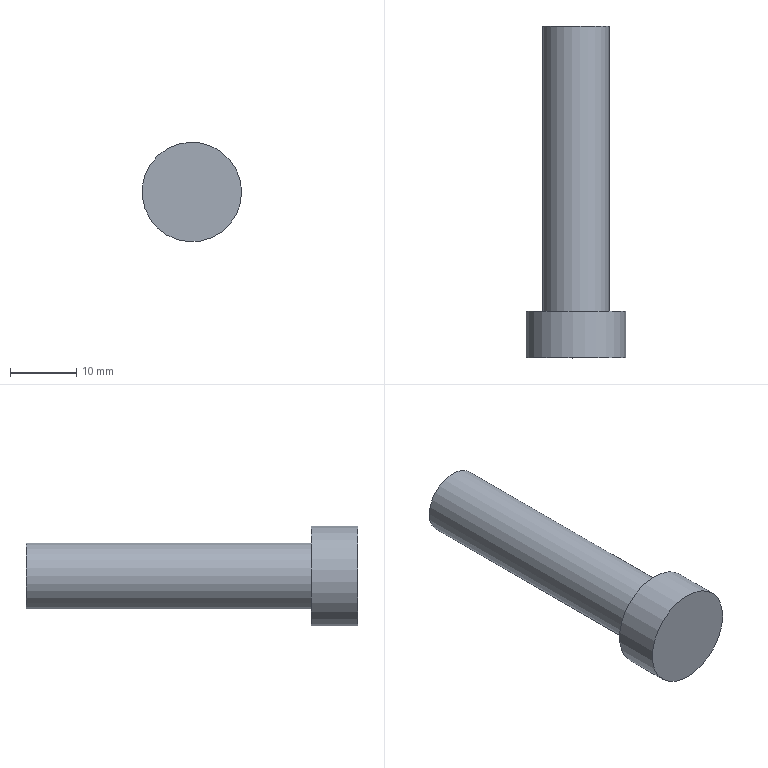Component | NX | LINK_PIN | 1 solid | 5 faces | box 15 x 50 x 15 mm | volume 4614 mm3 | plane 3 | cylinder 2 | commonest cylinder face diameters 10 x1 15 x1
STEP:
#1=CARTESIAN_POINT('',(0.,0.,0.));
#2=DIRECTION('',(0.,0.,1.));
#3=DIRECTION('',(1.,0.,0.));
#4=AXIS2_PLACEMENT_3D('',#1,#2,#3);
#5=CARTESIAN_POINT('',(12.507,-21.,-41.972));
#6=VERTEX_POINT('',#5);
#7=CARTESIAN_POINT('',(17.507,-21.,-41.994));
#8=DIRECTION('',(0.,-1.,0.));
#9=DIRECTION('',(-1.,0.,0.00428));
#10=AXIS2_PLACEMENT_3D('',#7,#8,#9);
#11=CIRCLE('',#10,5.);
#12=CARTESIAN_POINT('',(17.507,-28.,-41.994));
#13=DIRECTION('',(0.,1.,0.));
#14=DIRECTION('',(-1.,0.,0.00428));
#15=AXIS2_PLACEMENT_3D('',#12,#13,#14);
#16=CYLINDRICAL_SURFACE('',#15,5.);
#17=CARTESIAN_POINT('',(6.283,7.));
#18=DIRECTION('',(-1.,0.));
#19=VECTOR('',#18,1.);
#20=LINE('',#17,#19);
#21=(GEOMETRIC_REPRESENTATION_CONTEXT(2)PARAMETRIC_REPRESENTATION_CONTEXT()REPRESENTATION_CONTEXT('',''));
#22=DEFINITIONAL_REPRESENTATION('',(#20),#21);
#23=PCURVE('',#16,#22);
#24=CARTESIAN_POINT('',(17.507,-21.,-41.994));
#25=DIRECTION('',(0.,1.,0.));
#26=DIRECTION('',(-1.,0.,0.00428));
#27=AXIS2_PLACEMENT_3D('',#24,#25,#26);
#28=PLANE('',#27);
#29=CARTESIAN_POINT('',(5.,-0.));
#30=CARTESIAN_POINT('',(5.,-8.66));
#31=CARTESIAN_POINT('',(-2.5,-4.33));
#32=CARTESIAN_POINT('',(-10.,-0.));
#33=CARTESIAN_POINT('',(-2.5,4.33));
#34=CARTESIAN_POINT('',(5.,8.66));
#35=CARTESIAN_POINT('',(5.,-0.));
#36=(BOUNDED_CURVE()B_SPLINE_CURVE(2,(#29,#30,#31,#32,#33,#34,#35),.UNSPECIFIED.,.T.,.F.)B_SPLINE_CURVE_WITH_KNOTS((1,2,2,2,2,1),(-2.094,0.,2.094,4.189,6.283,8.378),.UNSPECIFIED.)CURVE()GEOMETRIC_REPRESENTATION_ITEM()RATIONAL_B_SPLINE_CURVE((1.,0.5,1.,0.5,1.,0.5,1.))REPRESENTATION_ITEM(''));
#37=(GEOMETRIC_REPRESENTATION_CONTEXT(2)PARAMETRIC_REPRESENTATION_CONTEXT()REPRESENTATION_CONTEXT('',''));
#38=DEFINITIONAL_REPRESENTATION('',(#36),#37);
#39=PCURVE('',#28,#38);
#40=SURFACE_CURVE('',#11,(#23,#39),.PCURVE_S1.);
#41=EDGE_CURVE('',#6,#6,#40,.T.);
#42=ORIENTED_EDGE('',*,*,#41,.F.);
#43=CARTESIAN_POINT('',(12.507,22.,-41.972));
#44=VERTEX_POINT('',#43);
#45=CARTESIAN_POINT('',(12.507,-21.,-41.972));
#46=CARTESIAN_POINT('',(12.507,22.,-41.972));
#47=B_SPLINE_CURVE_WITH_KNOTS('',1,(#45,#46),.UNSPECIFIED.,.F.,.F.,(2,2),(7.,50.),.PIECEWISE_BEZIER_KNOTS.);
#48=CARTESIAN_POINT('',(6.283,0.));
#49=DIRECTION('',(0.,1.));
#50=VECTOR('',#49,1.);
#51=LINE('',#48,#50);
#52=(GEOMETRIC_REPRESENTATION_CONTEXT(2)PARAMETRIC_REPRESENTATION_CONTEXT()REPRESENTATION_CONTEXT('',''));
#53=DEFINITIONAL_REPRESENTATION('',(#51),#52);
#54=PCURVE('',#16,#53);
#55=CARTESIAN_POINT('',(0.,0.));
#56=DIRECTION('',(0.,1.));
#57=VECTOR('',#56,1.);
#58=LINE('',#55,#57);
#59=(GEOMETRIC_REPRESENTATION_CONTEXT(2)PARAMETRIC_REPRESENTATION_CONTEXT()REPRESENTATION_CONTEXT('',''));
#60=DEFINITIONAL_REPRESENTATION('',(#58),#59);
#61=PCURVE('',#16,#60);
#62=SEAM_CURVE('',#47,(#54,#61),.PCURVE_S1.);
#63=EDGE_CURVE('',#6,#44,#62,.T.);
#64=ORIENTED_EDGE('',*,*,#63,.T.);
#65=CARTESIAN_POINT('',(22.506,22.,-42.015));
#66=VERTEX_POINT('',#65);
#67=CARTESIAN_POINT('',(17.507,22.,-41.994));
#68=DIRECTION('',(0.,1.,0.));
#69=DIRECTION('',(1.,0.,-0.00428));
#70=AXIS2_PLACEMENT_3D('',#67,#68,#69);
#71=CIRCLE('',#70,5.);
#72=CARTESIAN_POINT('',(3.142,50.));
#73=DIRECTION('',(1.,0.));
#74=VECTOR('',#73,1.);
#75=LINE('',#72,#74);
#76=(GEOMETRIC_REPRESENTATION_CONTEXT(2)PARAMETRIC_REPRESENTATION_CONTEXT()REPRESENTATION_CONTEXT('',''));
#77=DEFINITIONAL_REPRESENTATION('',(#75),#76);
#78=PCURVE('',#16,#77);
#79=CARTESIAN_POINT('',(17.507,22.,-41.994));
#80=DIRECTION('',(0.,1.,0.));
#81=DIRECTION('',(-1.,0.,0.00428));
#82=AXIS2_PLACEMENT_3D('',#79,#80,#81);
#83=PLANE('',#82);
#84=CARTESIAN_POINT('',(0.,0.));
#85=DIRECTION('',(-1.,0.));
#86=AXIS2_PLACEMENT_2D('',#84,#85);
#87=CIRCLE('',#86,5.);
#88=(GEOMETRIC_REPRESENTATION_CONTEXT(2)PARAMETRIC_REPRESENTATION_CONTEXT()REPRESENTATION_CONTEXT('',''));
#89=DEFINITIONAL_REPRESENTATION('',(#87),#88);
#90=PCURVE('',#83,#89);
#91=SURFACE_CURVE('',#71,(#78,#90),.PCURVE_S1.);
#92=EDGE_CURVE('',#66,#44,#91,.T.);
#93=ORIENTED_EDGE('',*,*,#92,.F.);
#94=CARTESIAN_POINT('',(17.507,22.,-41.994));
#95=DIRECTION('',(0.,1.,0.));
#96=DIRECTION('',(1.,0.,-0.00428));
#97=AXIS2_PLACEMENT_3D('',#94,#95,#96);
#98=CIRCLE('',#97,5.);
#99=CARTESIAN_POINT('',(-3.142,50.));
#100=DIRECTION('',(1.,0.));
#101=VECTOR('',#100,1.);
#102=LINE('',#99,#101);
#103=(GEOMETRIC_REPRESENTATION_CONTEXT(2)PARAMETRIC_REPRESENTATION_CONTEXT()REPRESENTATION_CONTEXT('',''));
#104=DEFINITIONAL_REPRESENTATION('',(#102),#103);
#105=PCURVE('',#16,#104);
#106=CARTESIAN_POINT('',(0.,0.));
#107=DIRECTION('',(-1.,0.));
#108=AXIS2_PLACEMENT_2D('',#106,#107);
#109=CIRCLE('',#108,5.);
#110=(GEOMETRIC_REPRESENTATION_CONTEXT(2)PARAMETRIC_REPRESENTATION_CONTEXT()REPRESENTATION_CONTEXT('',''));
#111=DEFINITIONAL_REPRESENTATION('',(#109),#110);
#112=PCURVE('',#83,#111);
#113=SURFACE_CURVE('',#98,(#105,#112),.PCURVE_S1.);
#114=EDGE_CURVE('',#44,#66,#113,.T.);
#115=ORIENTED_EDGE('',*,*,#114,.F.);
#116=ORIENTED_EDGE('',*,*,#63,.F.);
#117=EDGE_LOOP('',(#42,#64,#93,#115,#116));
#118=FACE_BOUND('',#117,.T.);
#119=ADVANCED_FACE('',(#118),#16,.T.);
#120=ORIENTED_EDGE('',*,*,#92,.T.);
#121=ORIENTED_EDGE('',*,*,#114,.T.);
#122=EDGE_LOOP('',(#120,#121));
#123=FACE_BOUND('',#122,.T.);
#124=ADVANCED_FACE('',(#123),#83,.T.);
#125=CARTESIAN_POINT('',(25.006,-28.,-42.026));
#126=VERTEX_POINT('',#125);
#127=CARTESIAN_POINT('',(17.507,-28.,-41.994));
#128=DIRECTION('',(0.,1.,0.));
#129=DIRECTION('',(1.,0.,-0.00428));
#130=AXIS2_PLACEMENT_3D('',#127,#128,#129);
#131=CIRCLE('',#130,7.5);
#132=CARTESIAN_POINT('',(17.507,-28.,-41.994));
#133=DIRECTION('',(0.,1.,0.));
#134=DIRECTION('',(-1.,0.,0.00428));
#135=AXIS2_PLACEMENT_3D('',#132,#133,#134);
#136=CYLINDRICAL_SURFACE('',#135,7.5);
#137=CARTESIAN_POINT('',(3.142,0.));
#138=DIRECTION('',(1.,0.));
#139=VECTOR('',#138,1.);
#140=LINE('',#137,#139);
#141=(GEOMETRIC_REPRESENTATION_CONTEXT(2)PARAMETRIC_REPRESENTATION_CONTEXT()REPRESENTATION_CONTEXT('',''));
#142=DEFINITIONAL_REPRESENTATION('',(#140),#141);
#143=PCURVE('',#136,#142);
#144=CARTESIAN_POINT('',(17.507,-28.,-41.994));
#145=DIRECTION('',(0.,1.,0.));
#146=DIRECTION('',(-1.,0.,0.00428));
#147=AXIS2_PLACEMENT_3D('',#144,#145,#146);
#148=PLANE('',#147);
#149=CARTESIAN_POINT('',(0.,0.));
#150=DIRECTION('',(-1.,0.));
#151=AXIS2_PLACEMENT_2D('',#149,#150);
#152=CIRCLE('',#151,7.5);
#153=(GEOMETRIC_REPRESENTATION_CONTEXT(2)PARAMETRIC_REPRESENTATION_CONTEXT()REPRESENTATION_CONTEXT('',''));
#154=DEFINITIONAL_REPRESENTATION('',(#152),#153);
#155=PCURVE('',#148,#154);
#156=SURFACE_CURVE('',#131,(#143,#155),.PCURVE_S1.);
#157=EDGE_CURVE('',#126,#126,#156,.T.);
#158=ORIENTED_EDGE('',*,*,#157,.T.);
#159=CARTESIAN_POINT('',(25.006,-21.,-42.026));
#160=VERTEX_POINT('',#159);
#161=CARTESIAN_POINT('',(25.006,-28.,-42.026));
#162=CARTESIAN_POINT('',(25.006,-21.,-42.026));
#163=B_SPLINE_CURVE_WITH_KNOTS('',1,(#161,#162),.UNSPECIFIED.,.F.,.F.,(2,2),(0.,7.),.PIECEWISE_BEZIER_KNOTS.);
#164=CARTESIAN_POINT('',(9.425,0.));
#165=DIRECTION('',(0.,1.));
#166=VECTOR('',#165,1.);
#167=LINE('',#164,#166);
#168=(GEOMETRIC_REPRESENTATION_CONTEXT(2)PARAMETRIC_REPRESENTATION_CONTEXT()REPRESENTATION_CONTEXT('',''));
#169=DEFINITIONAL_REPRESENTATION('',(#167),#168);
#170=PCURVE('',#136,#169);
#171=CARTESIAN_POINT('',(3.142,0.));
#172=DIRECTION('',(0.,1.));
#173=VECTOR('',#172,1.);
#174=LINE('',#171,#173);
#175=(GEOMETRIC_REPRESENTATION_CONTEXT(2)PARAMETRIC_REPRESENTATION_CONTEXT()REPRESENTATION_CONTEXT('',''));
#176=DEFINITIONAL_REPRESENTATION('',(#174),#175);
#177=PCURVE('',#136,#176);
#178=SEAM_CURVE('',#163,(#170,#177),.PCURVE_S1.);
#179=EDGE_CURVE('',#126,#160,#178,.T.);
#180=ORIENTED_EDGE('',*,*,#179,.T.);
#181=CARTESIAN_POINT('',(17.507,-21.,-41.994));
#182=DIRECTION('',(0.,1.,0.));
#183=DIRECTION('',(1.,0.,-0.00428));
#184=AXIS2_PLACEMENT_3D('',#181,#182,#183);
#185=CIRCLE('',#184,7.5);
#186=CARTESIAN_POINT('',(3.142,7.));
#187=DIRECTION('',(1.,0.));
#188=VECTOR('',#187,1.);
#189=LINE('',#186,#188);
#190=(GEOMETRIC_REPRESENTATION_CONTEXT(2)PARAMETRIC_REPRESENTATION_CONTEXT()REPRESENTATION_CONTEXT('',''));
#191=DEFINITIONAL_REPRESENTATION('',(#189),#190);
#192=PCURVE('',#136,#191);
#193=CARTESIAN_POINT('',(0.,0.));
#194=DIRECTION('',(-1.,0.));
#195=AXIS2_PLACEMENT_2D('',#193,#194);
#196=CIRCLE('',#195,7.5);
#197=(GEOMETRIC_REPRESENTATION_CONTEXT(2)PARAMETRIC_REPRESENTATION_CONTEXT()REPRESENTATION_CONTEXT('',''));
#198=DEFINITIONAL_REPRESENTATION('',(#196),#197);
#199=PCURVE('',#28,#198);
#200=SURFACE_CURVE('',#185,(#192,#199),.PCURVE_S1.);
#201=EDGE_CURVE('',#160,#160,#200,.T.);
#202=ORIENTED_EDGE('',*,*,#201,.F.);
#203=ORIENTED_EDGE('',*,*,#179,.F.);
#204=EDGE_LOOP('',(#158,#180,#202,#203));
#205=FACE_BOUND('',#204,.T.);
#206=ADVANCED_FACE('',(#205),#136,.T.);
#207=ORIENTED_EDGE('',*,*,#41,.T.);
#208=EDGE_LOOP('',(#207));
#209=FACE_BOUND('',#208,.T.);
#210=ORIENTED_EDGE('',*,*,#201,.T.);
#211=EDGE_LOOP('',(#210));
#212=FACE_BOUND('',#211,.T.);
#213=ADVANCED_FACE('',(#209,#212),#28,.T.);
#214=ORIENTED_EDGE('',*,*,#157,.F.);
#215=EDGE_LOOP('',(#214));
#216=FACE_BOUND('',#215,.T.);
#217=ADVANCED_FACE('',(#216),#148,.F.);
#218=CLOSED_SHELL('',(#119,#124,#206,#213,#217));
#219=MANIFOLD_SOLID_BREP('',#218);
#220=(LENGTH_UNIT()NAMED_UNIT(*)SI_UNIT(.MILLI.,.METRE.));
#221=UNCERTAINTY_MEASURE_WITH_UNIT(LENGTH_MEASURE(0.000005),#220,'','');
#222=(NAMED_UNIT(*)PLANE_ANGLE_UNIT()SI_UNIT($,.RADIAN.));
#223=(NAMED_UNIT(*)SI_UNIT($,.STERADIAN.)SOLID_ANGLE_UNIT());
#224=(GEOMETRIC_REPRESENTATION_CONTEXT(3)GLOBAL_UNCERTAINTY_ASSIGNED_CONTEXT((#221))GLOBAL_UNIT_ASSIGNED_CONTEXT((#220,#222,#223))REPRESENTATION_CONTEXT('',''));
#225=ADVANCED_BREP_SHAPE_REPRESENTATION('',(#4,#219),#224);